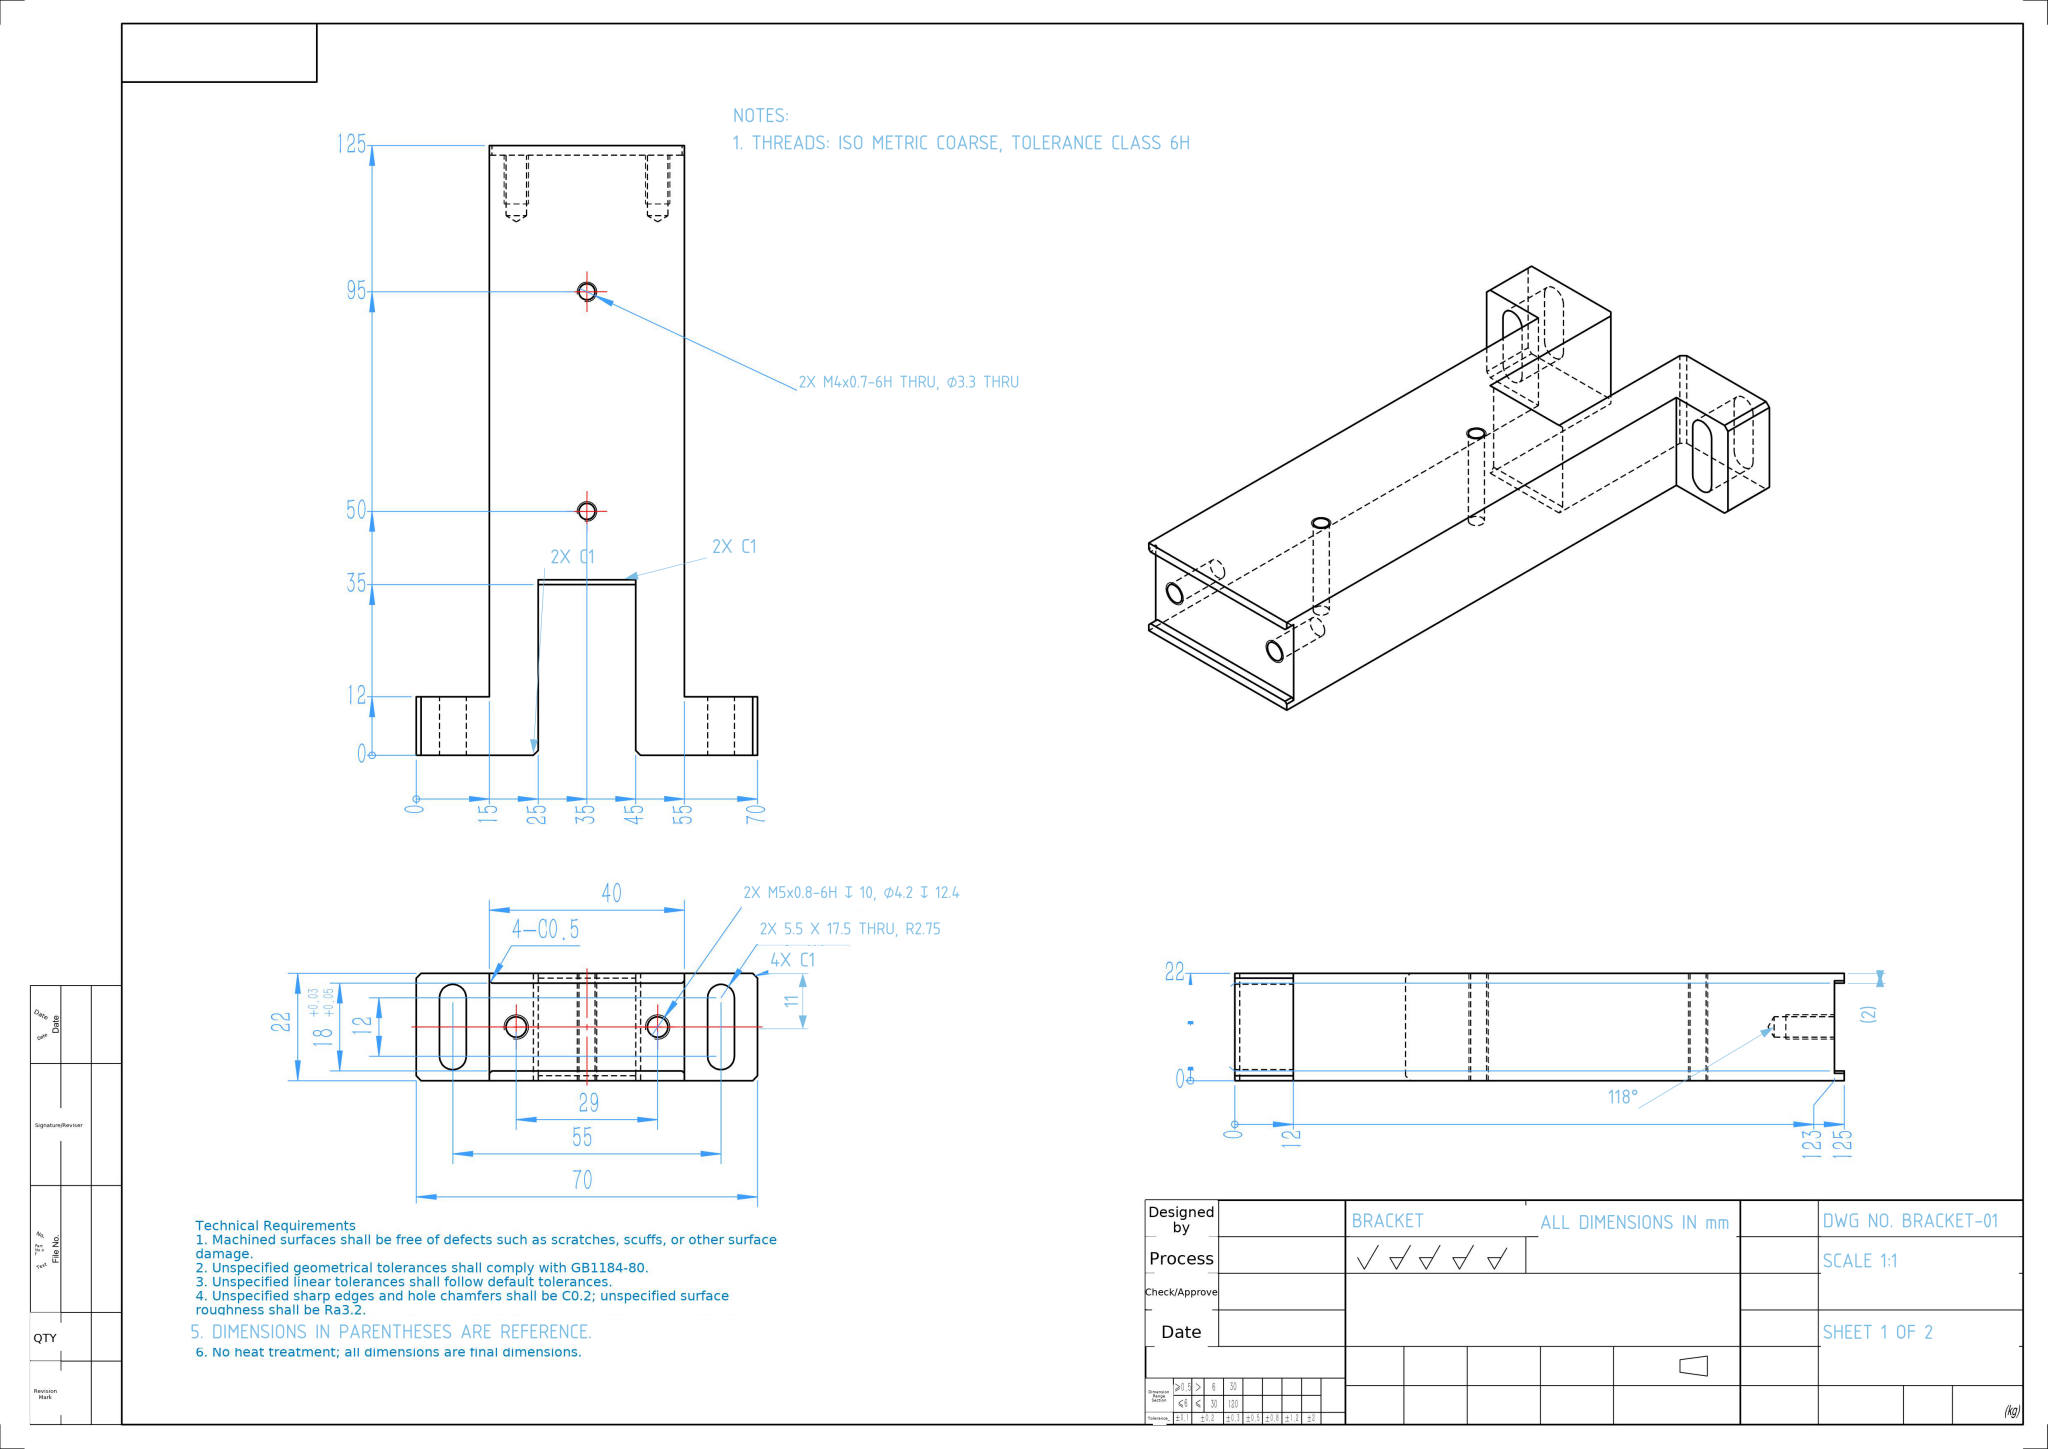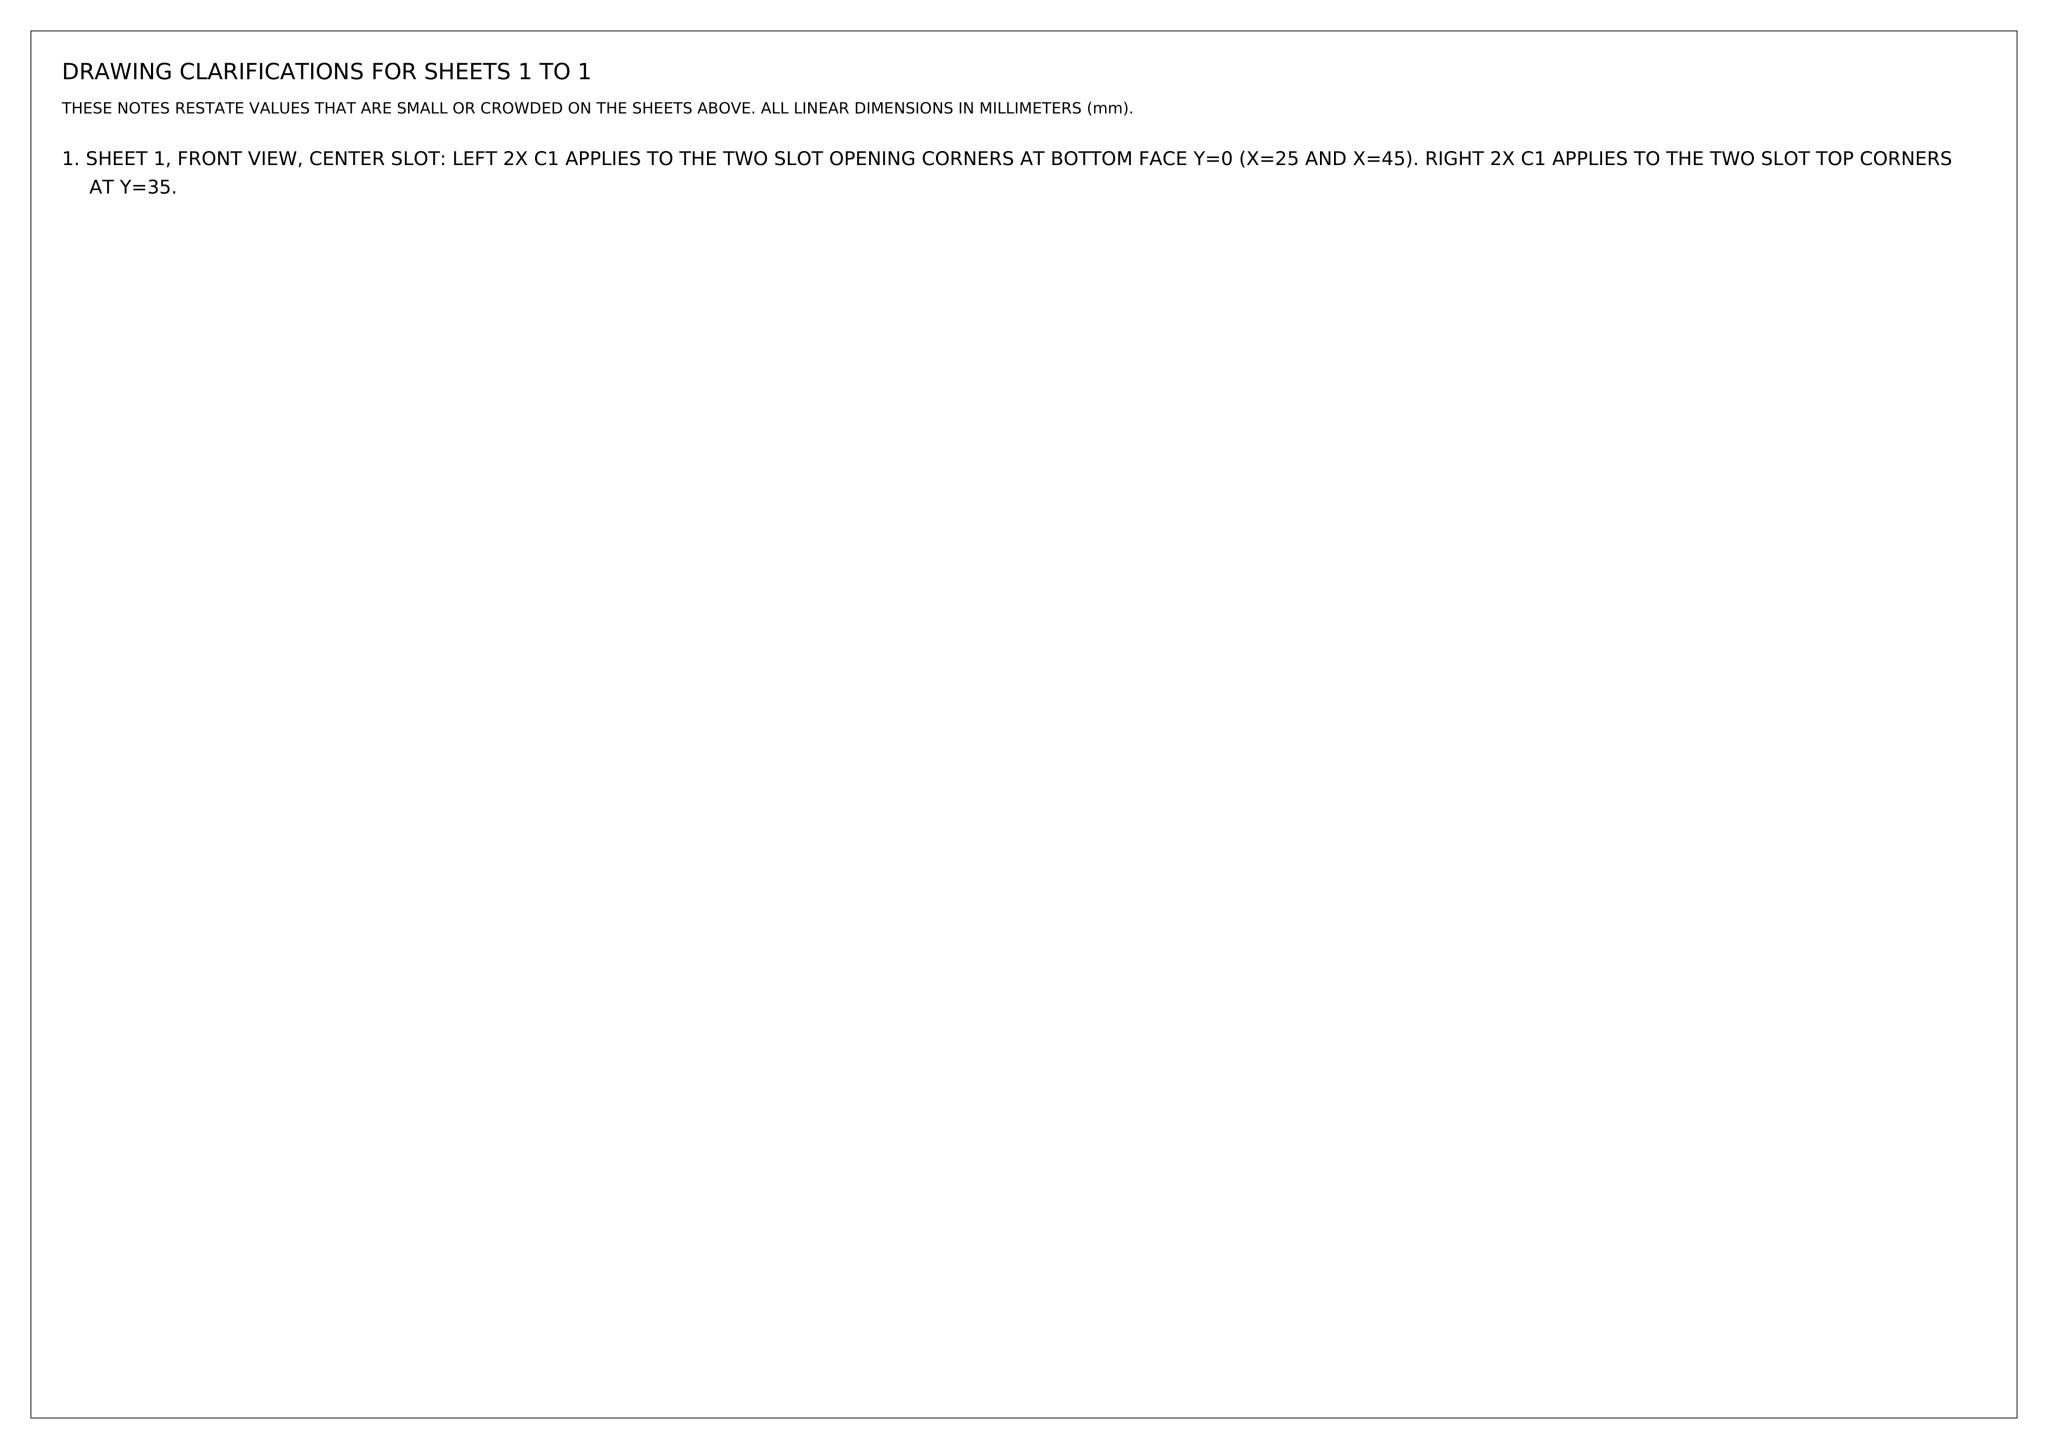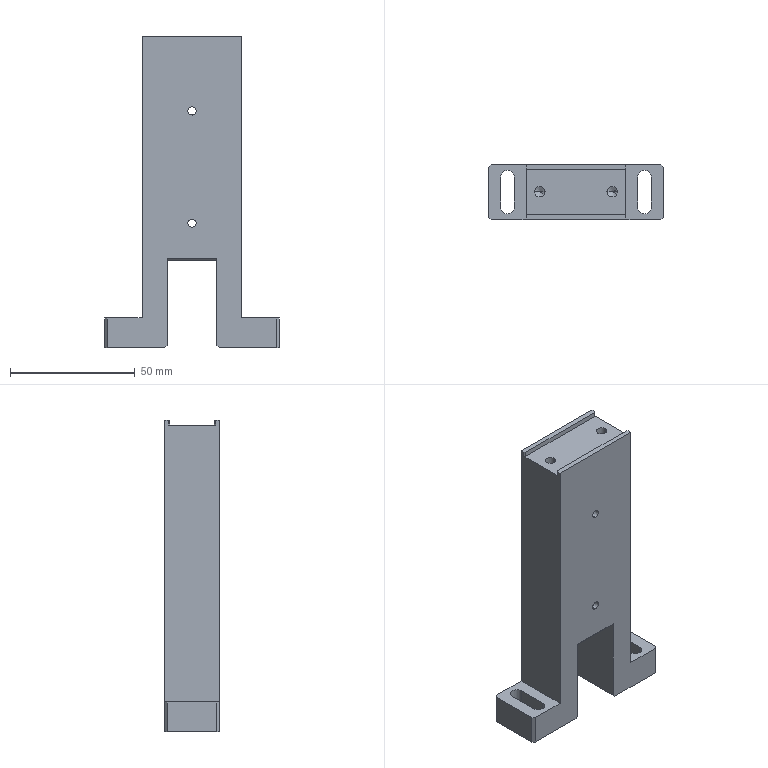Part | NX | mm | 1 solid | 50 faces | box 70 x 22 x 125 mm | volume 98127 mm3 | plane 34 | cylinder 12 | cone 4 | commonest cylinder face diameters 3.3 x4 4.2 x4 5.5 x4